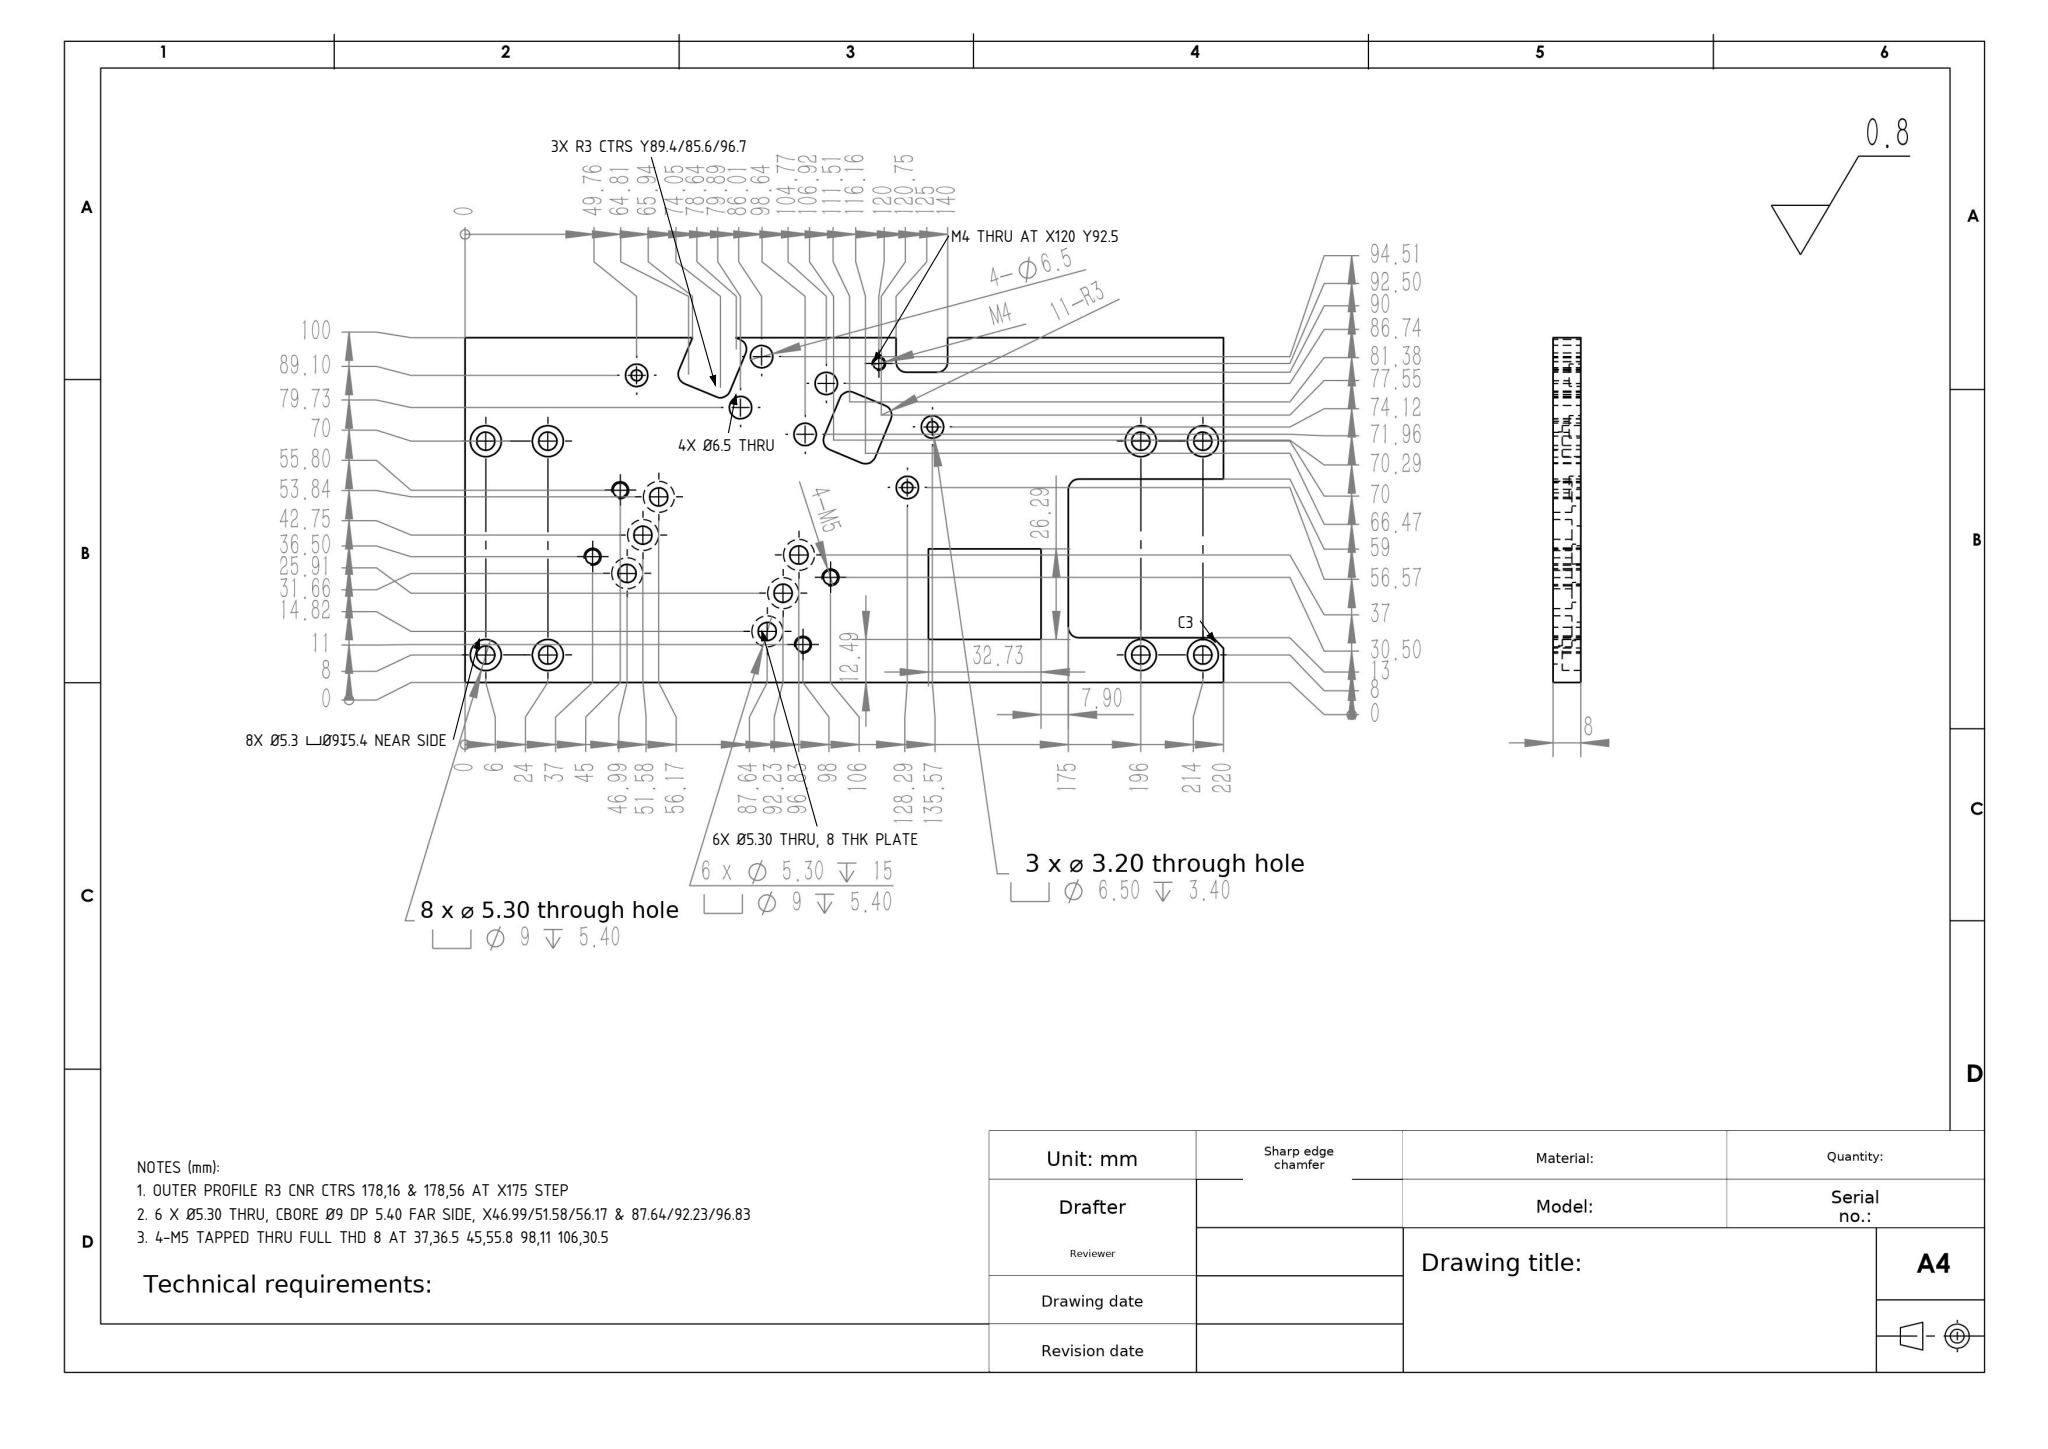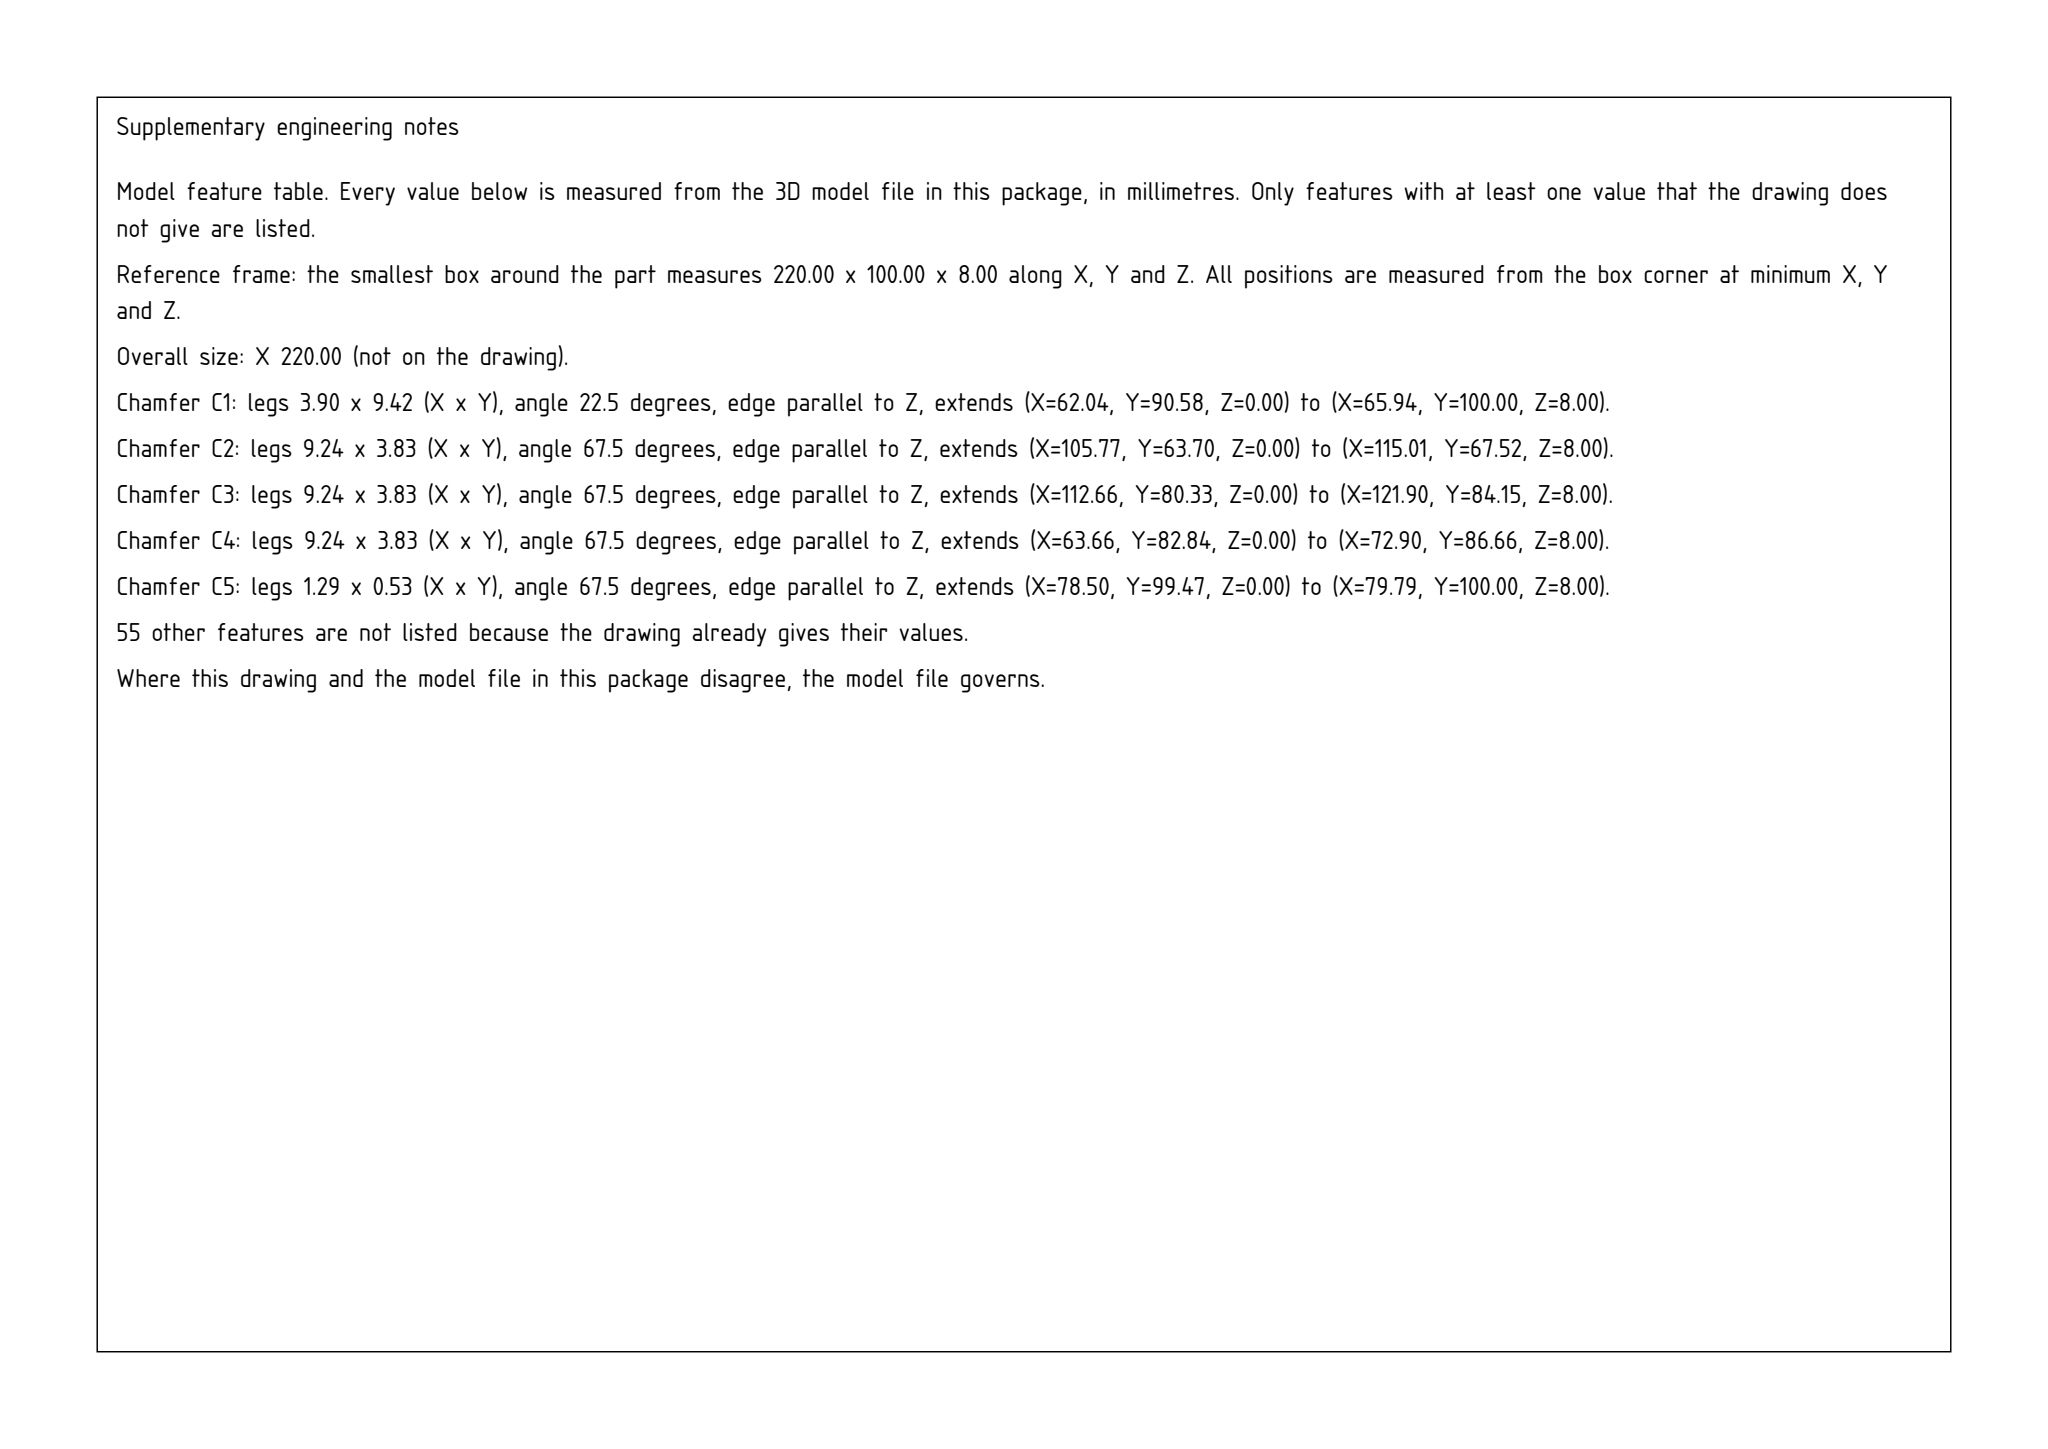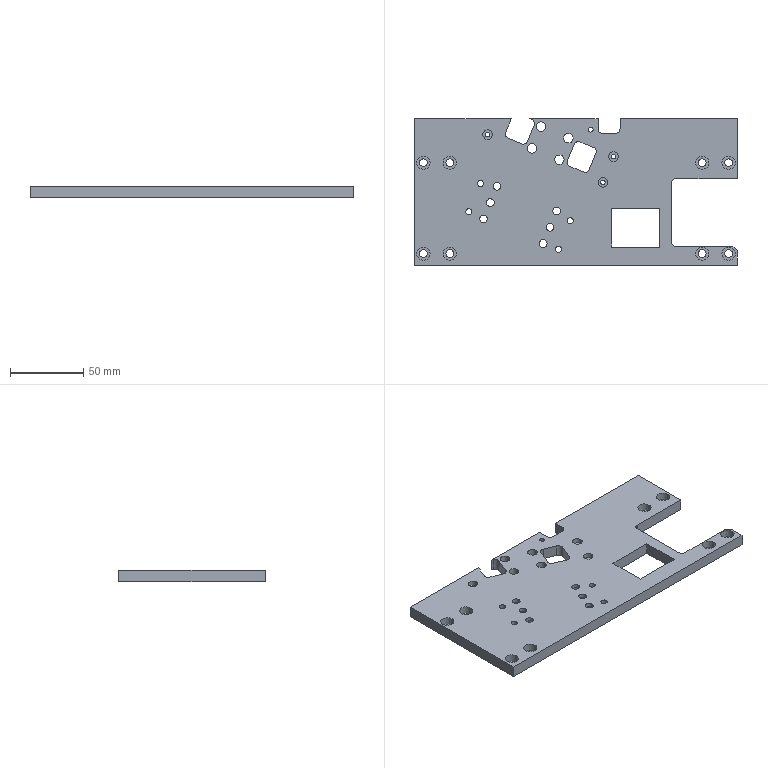Part | SolidWorks | mm | 1 solid | 144 faces | box 220 x 100 x 8 mm | volume 139471 mm3 | cylinder 99 | plane 45 | commonest cylinder face diameters 9 x28 5.3 x28 6.5 x14 6 x13 4.2 x8 3.2 x6 3.3 x2
Drawing notes:
OUTER PROFILE R3 CNR CTRS 178,16 & 178,56 AT X175 STEP | from the solid: Ø6 L=8 at (178,16)(178,56); X plane 175, Y planes 13/59
8 X Ø5.30 THRU, CBORE Ø9 DP 5.40 NEAR SIDE, AT X6/24/196/214 | from the solid: Ø5.3 L=2.6 + Ø9 L=5.4; z-plane 2.60 count 8
6 X Ø5.30 THRU, CBORE Ø9 DP 5.40 FAR SIDE, X46.99/51.58/56.17 & 87.64/92.23/96.83 | from the solid: Ø5.3 L=2.6 + Ø9 L=5.4; z-plane 5.40 count 6
4 X Ø6.5 THRU AT 79.89,79.73 86.01,94.51 98.64,71.96 104.77,86.74 | from the solid: Ø6.5 z-holes L=8 at those positions
4-M5 TAPPED THRU FULL THD 8 AT 37,36.5 45,55.8 98,11 106,30.5 | from the solid: Ø4.2 z-holes L=8 at those positions
1-M4 TAPPED THRU FULL THD 8 AT 120,92.5 | from the solid: Ø3.3 z-hole L=8 at (120,92.5)
UPPER LH TOP CUTOUT: R3 CTRS Y 89.40, 85.60, 96.70 FM BTM EDGE | from the solid: R3 arcs (dia 6, z-axis) at [64.8,89.4], [74.1,85.6], [78.6,96.7]; cutout breaks top edge y=100 between x=65.9 and x=78.5
LWR RH CORNER C3: X217,Y13 TO X220,Y10 FM LH/BTM EDGES | from the solid: inclined plane 45/45/90, bbox_from [217,10,0], size [3,3,8]; face y=13 ends x=217, face x=220 ends y=10
6 X Ø5.30 THRU, CBORE Ø9 DP 5.40 (NOT DP 15) - PLATE 8 THK | from the solid: Ø5.3 holes at [47,31.7],[51.6,42.7],[56.2,53.8],[87.6,14.8],[92.2,25.9],[96.8,37] run z 5.4-8.0 with Ø9 cbore z 0-5.4; plate z 0-8
build123d program:
from build123d import *

# Parameters (mm, degrees)
SKETCH1_W                                       = 220
SKETCH1_H                                       = 100
BOSS_EXTRUDE1_DEPTH                             = 8
M5_HEX_SOCKET_HEAD_CAP_SCREW_CBORE1_D           = 5.3
M5_HEX_SOCKET_HEAD_CAP_SCREW_CBORE1_DEPTH       = 15
M5_HEX_SOCKET_HEAD_CAP_SCREW_CBORE1_CBORE_D     = 9
M5_HEX_SOCKET_HEAD_CAP_SCREW_CBORE1_CBORE_DEPTH = 5.4
M5_HEX_SOCKET_HEAD_CAP_SCREW_CBORE1_TIP         = 1.592
SKETCH6_W                                       = 15
SKETCH6_H                                       = 10
CUT_EXTRUDE2_DEPTH                              = 242.793
M5_HEX_SOCKET_HEAD_CAP_SCREW_CBORE2_D           = 5.3
M5_HEX_SOCKET_HEAD_CAP_SCREW_CBORE2_CBORE_D     = 9
M5_HEX_SOCKET_HEAD_CAP_SCREW_CBORE2_CBORE_DEPTH = 5.4
FILLET1_R                                       = 3
CUT_EXTRUDE3_DEPTH                              = 242.793
F_6_5_6_5_DIAMETER_HOLE1_D                      = 6.5
F_6_5_6_5_DIAMETER_HOLE1_DEPTH                  = 10
F_6_5_6_5_DIAMETER_HOLE1_TIP                    = 1.953
FILLET2_R                                       = 3
CUT_EXTRUDE4_DEPTH                              = 242.793
M4_TAPPED_HOLE1_D                               = 3.3
M3_HEX_SOCKET_HEAD_CAP_SCREW_CBORE1_D           = 3.2
M3_HEX_SOCKET_HEAD_CAP_SCREW_CBORE1_CBORE_D     = 6.5
M3_HEX_SOCKET_HEAD_CAP_SCREW_CBORE1_CBORE_DEPTH = 3.4
M5_TAPPED_HOLE1_D                               = 4.2
SKETCH18_W                                      = 45
SKETCH18_H                                      = 46
CUT_EXTRUDE6_DEPTH                              = 242.793
FILLET3_R                                       = 3
CHAMFER1_SIZE                                   = 3
SKETCH19_W                                      = 32.727
SKETCH19_H                                      = 26.286
CUT_EXTRUDE7_DEPTH                              = 66


with BuildPart() as part:
    # Sketch1 → Boss-Extrude1 (new body)
    with BuildSketch(Plane.XY):
        with Locations((110, 50)):
            Rectangle(SKETCH1_W, SKETCH1_H)
    extrude(amount=BOSS_EXTRUDE1_DEPTH)

    # M5 Hex Socket Head Cap Screw CBORE1
    with Locations(Plane(origin=(87.641, 14.824, 0), x_dir=(-1, 0, 0), z_dir=(0, 0, -1))):
        with Locations((0, 0), (-4.592, 11.087), (-9.184, 22.173), (31.466, 39.011), (36.058, 27.925), (40.651, 16.838)):
            CounterBoreHole(M5_HEX_SOCKET_HEAD_CAP_SCREW_CBORE1_D / 2, M5_HEX_SOCKET_HEAD_CAP_SCREW_CBORE1_CBORE_D / 2, M5_HEX_SOCKET_HEAD_CAP_SCREW_CBORE1_CBORE_DEPTH, depth=M5_HEX_SOCKET_HEAD_CAP_SCREW_CBORE1_DEPTH)
            with Locations((0, 0, -(M5_HEX_SOCKET_HEAD_CAP_SCREW_CBORE1_DEPTH + M5_HEX_SOCKET_HEAD_CAP_SCREW_CBORE1_TIP / 2))):  # 118° drill point
                Cone(0, M5_HEX_SOCKET_HEAD_CAP_SCREW_CBORE1_D / 2, M5_HEX_SOCKET_HEAD_CAP_SCREW_CBORE1_TIP, mode=Mode.SUBTRACT)

    # Sketch6 → Cut-Extrude2 (cut, through all)
    with BuildSketch(Plane.XY.offset(8)):
        with Locations((132.5, 95)):
            Rectangle(SKETCH6_W, SKETCH6_H)
    extrude(amount=-CUT_EXTRUDE2_DEPTH, mode=Mode.SUBTRACT)

    # M5 Hex Socket Head Cap Screw CBORE2 (through all)
    with Locations(Plane(origin=(24, 70, 8), x_dir=(1, 0, 0), z_dir=(0, 0, 1))):
        with Locations((0, 0), (-18, 0), (0, -62), (-18, -62), (172, -62), (190, -62), (190, 0), (172, 0)):
            CounterBoreHole(M5_HEX_SOCKET_HEAD_CAP_SCREW_CBORE2_D / 2, M5_HEX_SOCKET_HEAD_CAP_SCREW_CBORE2_CBORE_D / 2, M5_HEX_SOCKET_HEAD_CAP_SCREW_CBORE2_CBORE_DEPTH)

    # Fillet1
    fillet1_edges = [part.edges().sort_by_distance(p)[0] for p in [
        (125, 90, 4),
        (140, 90, 4),
    ]]
    fillet(fillet1_edges, radius=FILLET1_R)

    # Sketch8 → Cut-Extrude3 (cut, through all)
    with BuildSketch(Plane.XY.offset(8)):
        Polygon((124.67, 79.177), (109.888, 85.3), (103, 68.67), (117.782, 62.547), align=None)
    extrude(amount=-CUT_EXTRUDE3_DEPTH, mode=Mode.SUBTRACT)

    # 6.5 _6.5_ Diameter Hole1
    with Locations(Plane(origin=(98.644, 71.963, 0), x_dir=(-1, 0, 0), z_dir=(0, 0, -1))):
        with Locations((0, 0), (18.755, 7.768), (-6.123, 14.782), (12.632, 22.551)):
            Hole(F_6_5_6_5_DIAMETER_HOLE1_D / 2, depth=F_6_5_6_5_DIAMETER_HOLE1_DEPTH)
            with Locations((0, 0, -(F_6_5_6_5_DIAMETER_HOLE1_DEPTH + F_6_5_6_5_DIAMETER_HOLE1_TIP / 2))):  # 118° drill point
                Cone(0, F_6_5_6_5_DIAMETER_HOLE1_D / 2, F_6_5_6_5_DIAMETER_HOLE1_TIP, mode=Mode.SUBTRACT)

    # Fillet2
    fillet2_edges = [part.edges().sort_by_distance(p)[0] for p in [
        (124.67, 79.177, 4),
        (117.782, 62.547, 4),
        (103, 68.67, 4),
        (109.888, 85.3, 4),
    ]]
    fillet(fillet2_edges, radius=FILLET2_R)

    # Sketch12 → Cut-Extrude4 (cut, through all)
    with BuildSketch(Plane(origin=(0, 0, 0), x_dir=(-1, 0, 0), z_dir=(0, 0, -1))):
        with BuildLine():
            Line((-72.902, 82.837), (-63.663, 86.664))
            ThreePointArc((-63.663, 86.664), (-62.04, 88.287), (-62.04, 90.584))
            Line((-62.04, 90.584), (-66.632, 101.67))
            ThreePointArc((-66.632, 101.67), (-68.256, 103.294), (-70.552, 103.294))
            Line((-70.552, 103.294), (-79.791, 99.467))
            ThreePointArc((-79.791, 99.467), (-81.414, 97.843), (-81.414, 95.547))
            Line((-81.414, 95.547), (-76.822, 84.461))
            ThreePointArc((-76.822, 84.461), (-75.198, 82.837), (-72.902, 82.837))
        make_face()
    extrude(amount=-CUT_EXTRUDE4_DEPTH, mode=Mode.SUBTRACT)

    # M4 Tapped Hole1 (through all)
    with Locations(Plane(origin=(120, 92.5, 0), x_dir=(-1, 0, 0), z_dir=(0, 0, -1))):
        with Locations((0, 0)):
            Hole(M4_TAPPED_HOLE1_D / 2)

    # M3 Hex Socket Head Cap Screw CBORE1 (through all)
    with Locations(Plane(origin=(135.566, 74.123, 8), x_dir=(1, 0, 0), z_dir=(0, 0, 1))):
        with Locations((0, 0), (-7.271, -17.554), (-85.801, 14.974)):
            CounterBoreHole(M3_HEX_SOCKET_HEAD_CAP_SCREW_CBORE1_D / 2, M3_HEX_SOCKET_HEAD_CAP_SCREW_CBORE1_CBORE_D / 2, M3_HEX_SOCKET_HEAD_CAP_SCREW_CBORE1_CBORE_DEPTH)

    # M5 Tapped Hole1 (through all)
    with Locations(Plane(origin=(45, 55.8, 8), x_dir=(1, 0, 0), z_dir=(0, 0, 1))):
        with Locations((0, 0), (-8, -19.3), (53, -44.8), (61, -25.3)):
            Hole(M5_TAPPED_HOLE1_D / 2)

    # Sketch18 → Cut-Extrude6 (cut, through all)
    with BuildSketch(Plane.XY.offset(8)):
        with Locations((197.5, 36)):
            Rectangle(SKETCH18_W, SKETCH18_H)
    extrude(amount=-CUT_EXTRUDE6_DEPTH, mode=Mode.SUBTRACT)

    # Fillet3
    fillet3_edges = [part.edges().sort_by_distance(p)[0] for p in [
        (175, 13, 4),
        (175, 59, 4),
    ]]
    fillet(fillet3_edges, radius=FILLET3_R)

    # Chamfer1
    chamfer1_edges = [part.edges().sort_by_distance(p)[0] for p in [
        (220, 13, 4),
    ]]
    chamfer(chamfer1_edges, length=CHAMFER1_SIZE)

    # Sketch19 → Cut-Extrude7 (cut)
    with BuildSketch(Plane.XY.offset(8)):
        with Locations((150.735, 25.629)):
            Rectangle(SKETCH19_W, SKETCH19_H)
    extrude(amount=-CUT_EXTRUDE7_DEPTH, mode=Mode.SUBTRACT)


solid = part.part